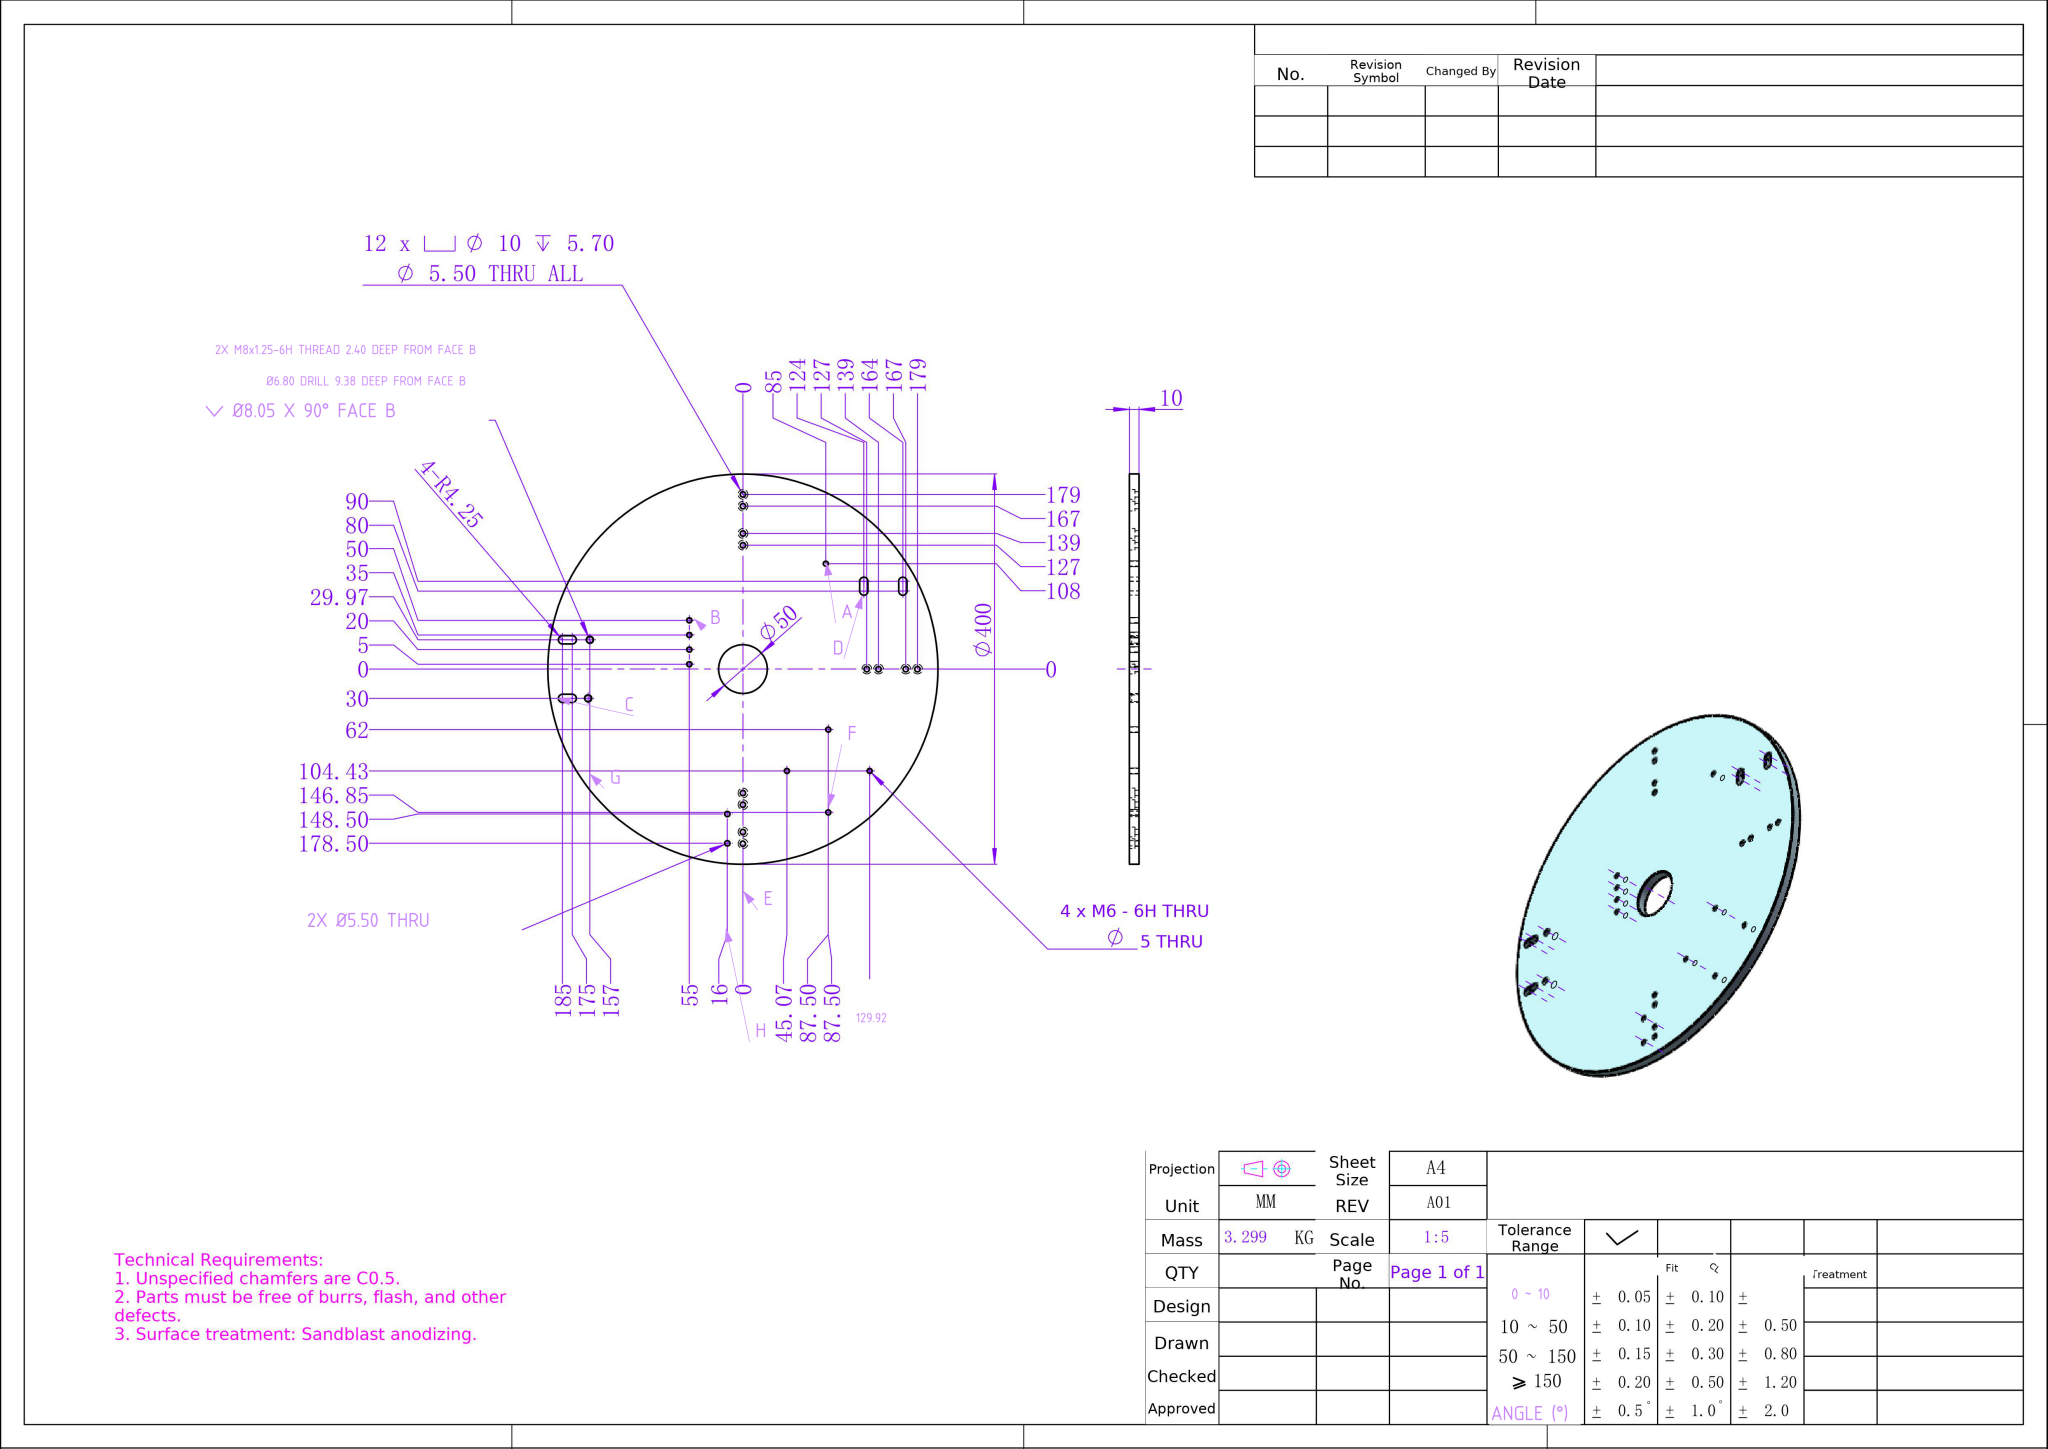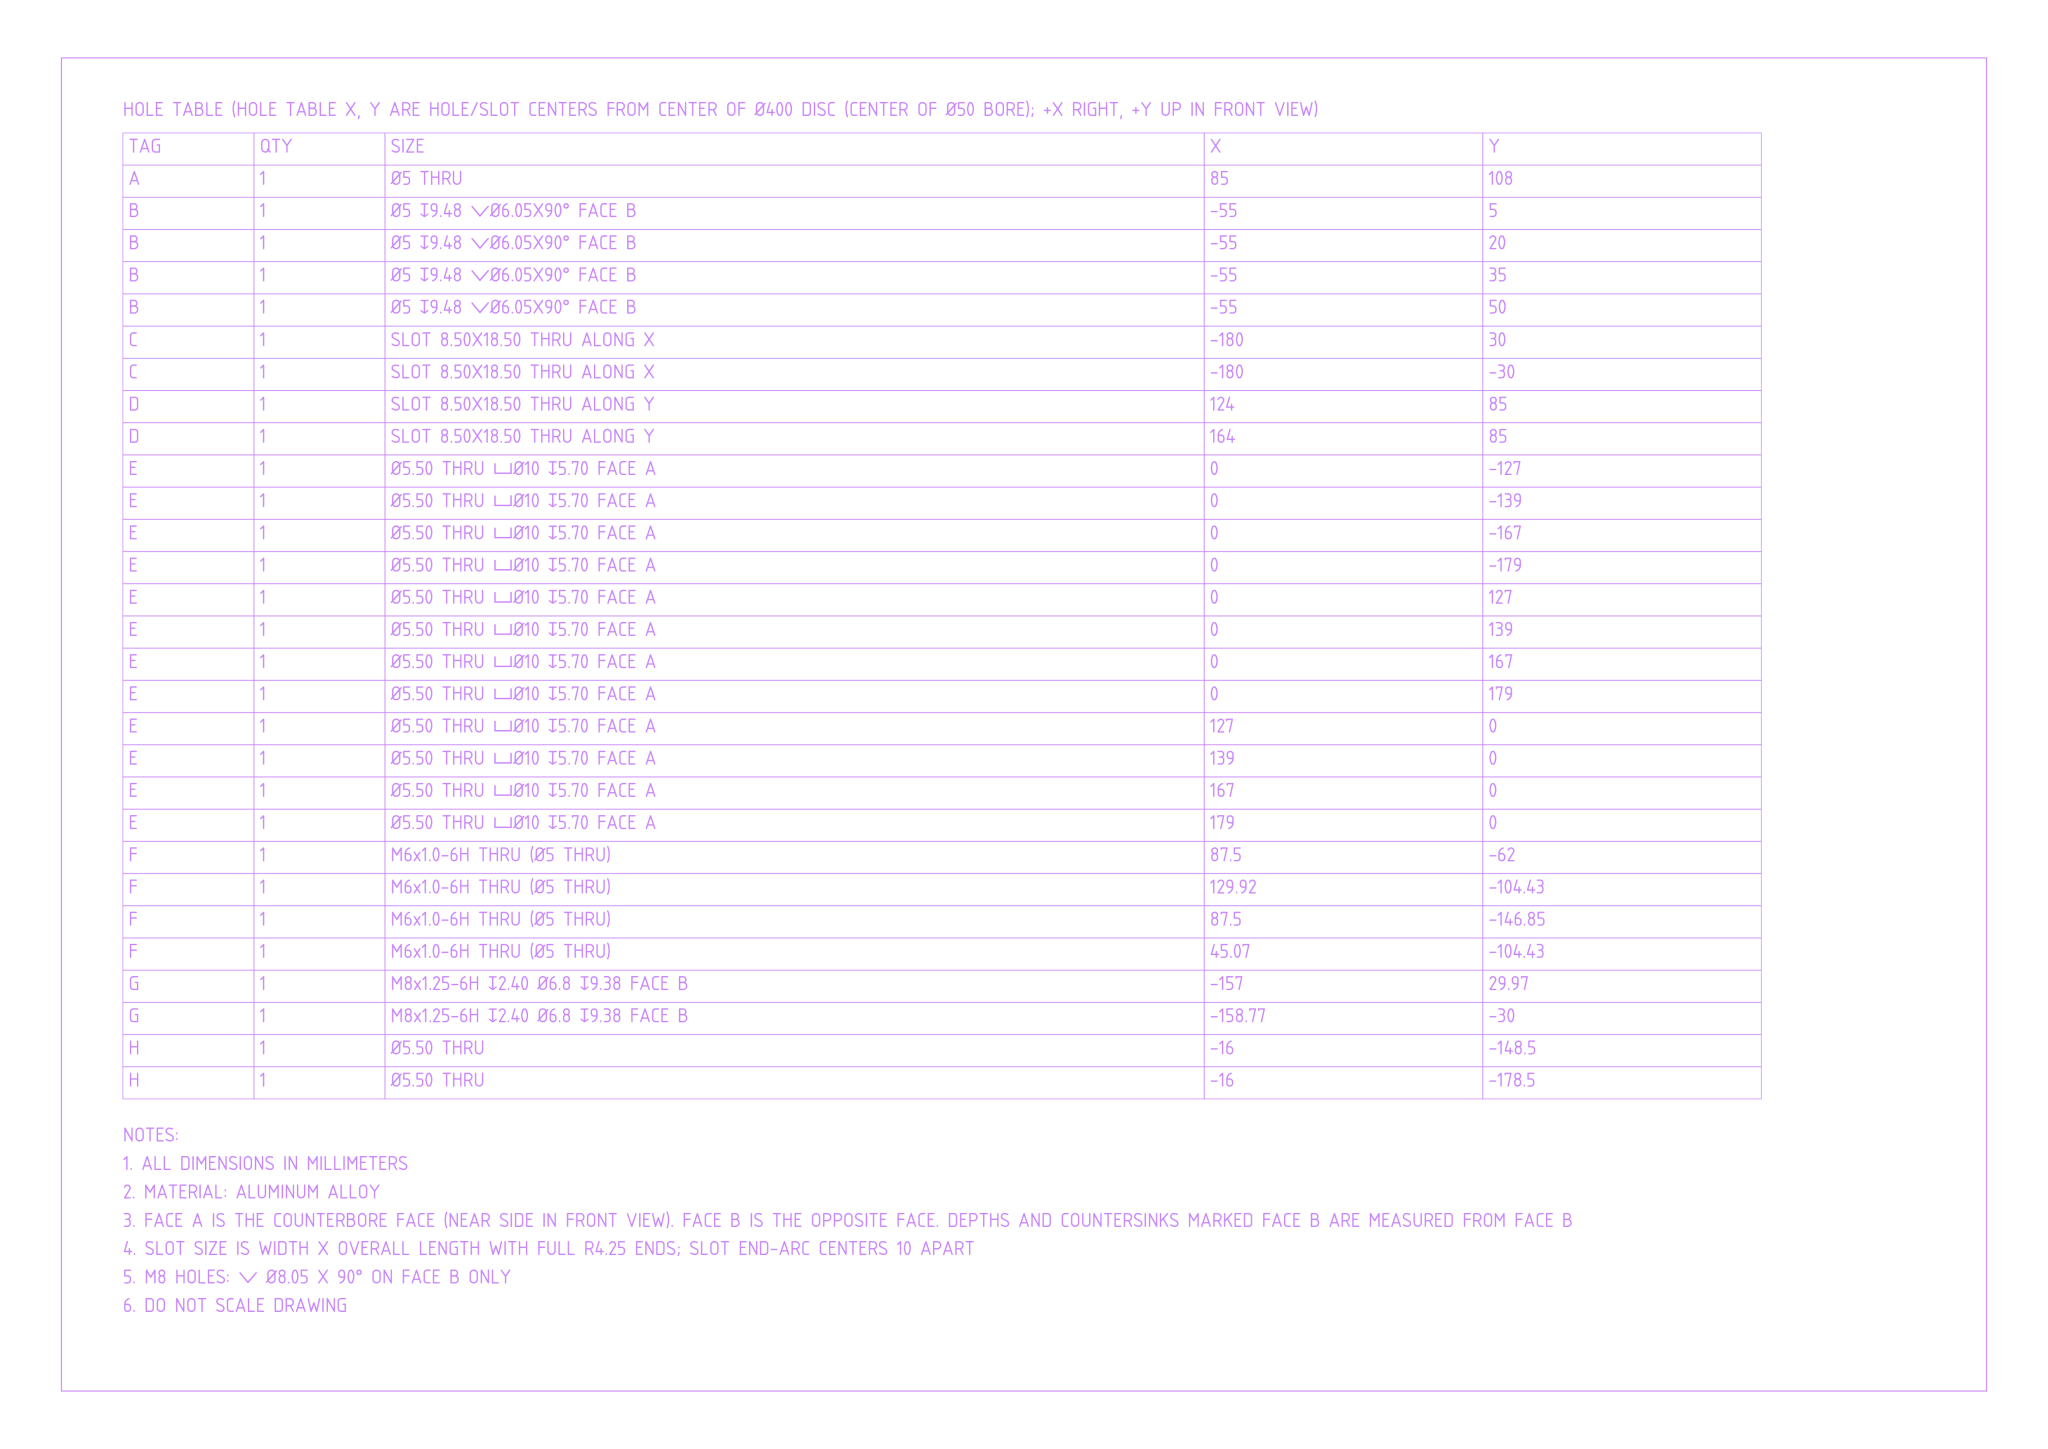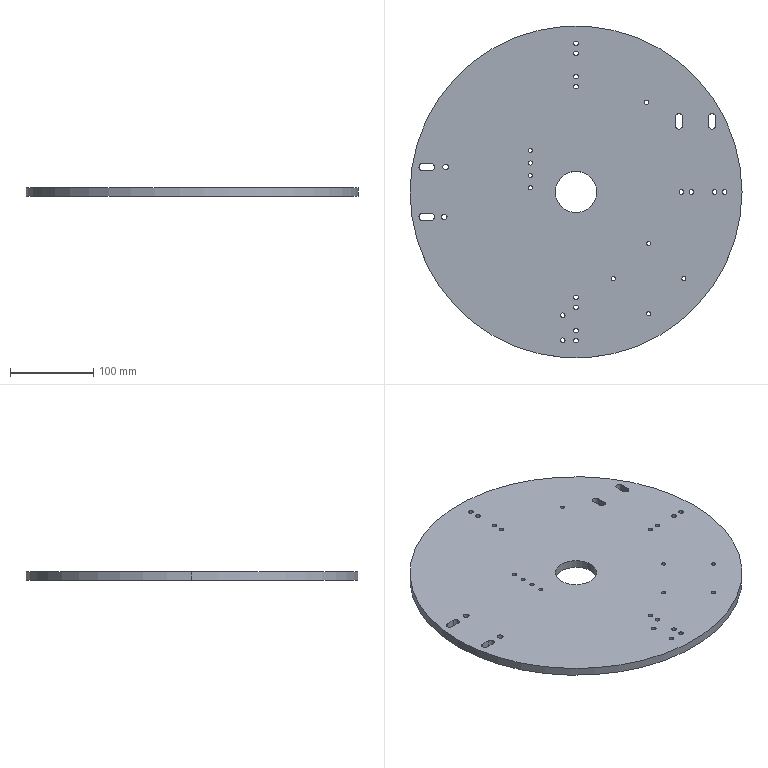Part | NX | mm | 1 solid | 122 faces | box 400 x 400 x 10 mm | volume 1221747 mm3 | cylinder 88 | plane 22 | cone 12 | commonest cylinder face diameters 5.5 x28 10 x24 5 x18 8.5 x10 6.8 x4 50 x2 400 x2